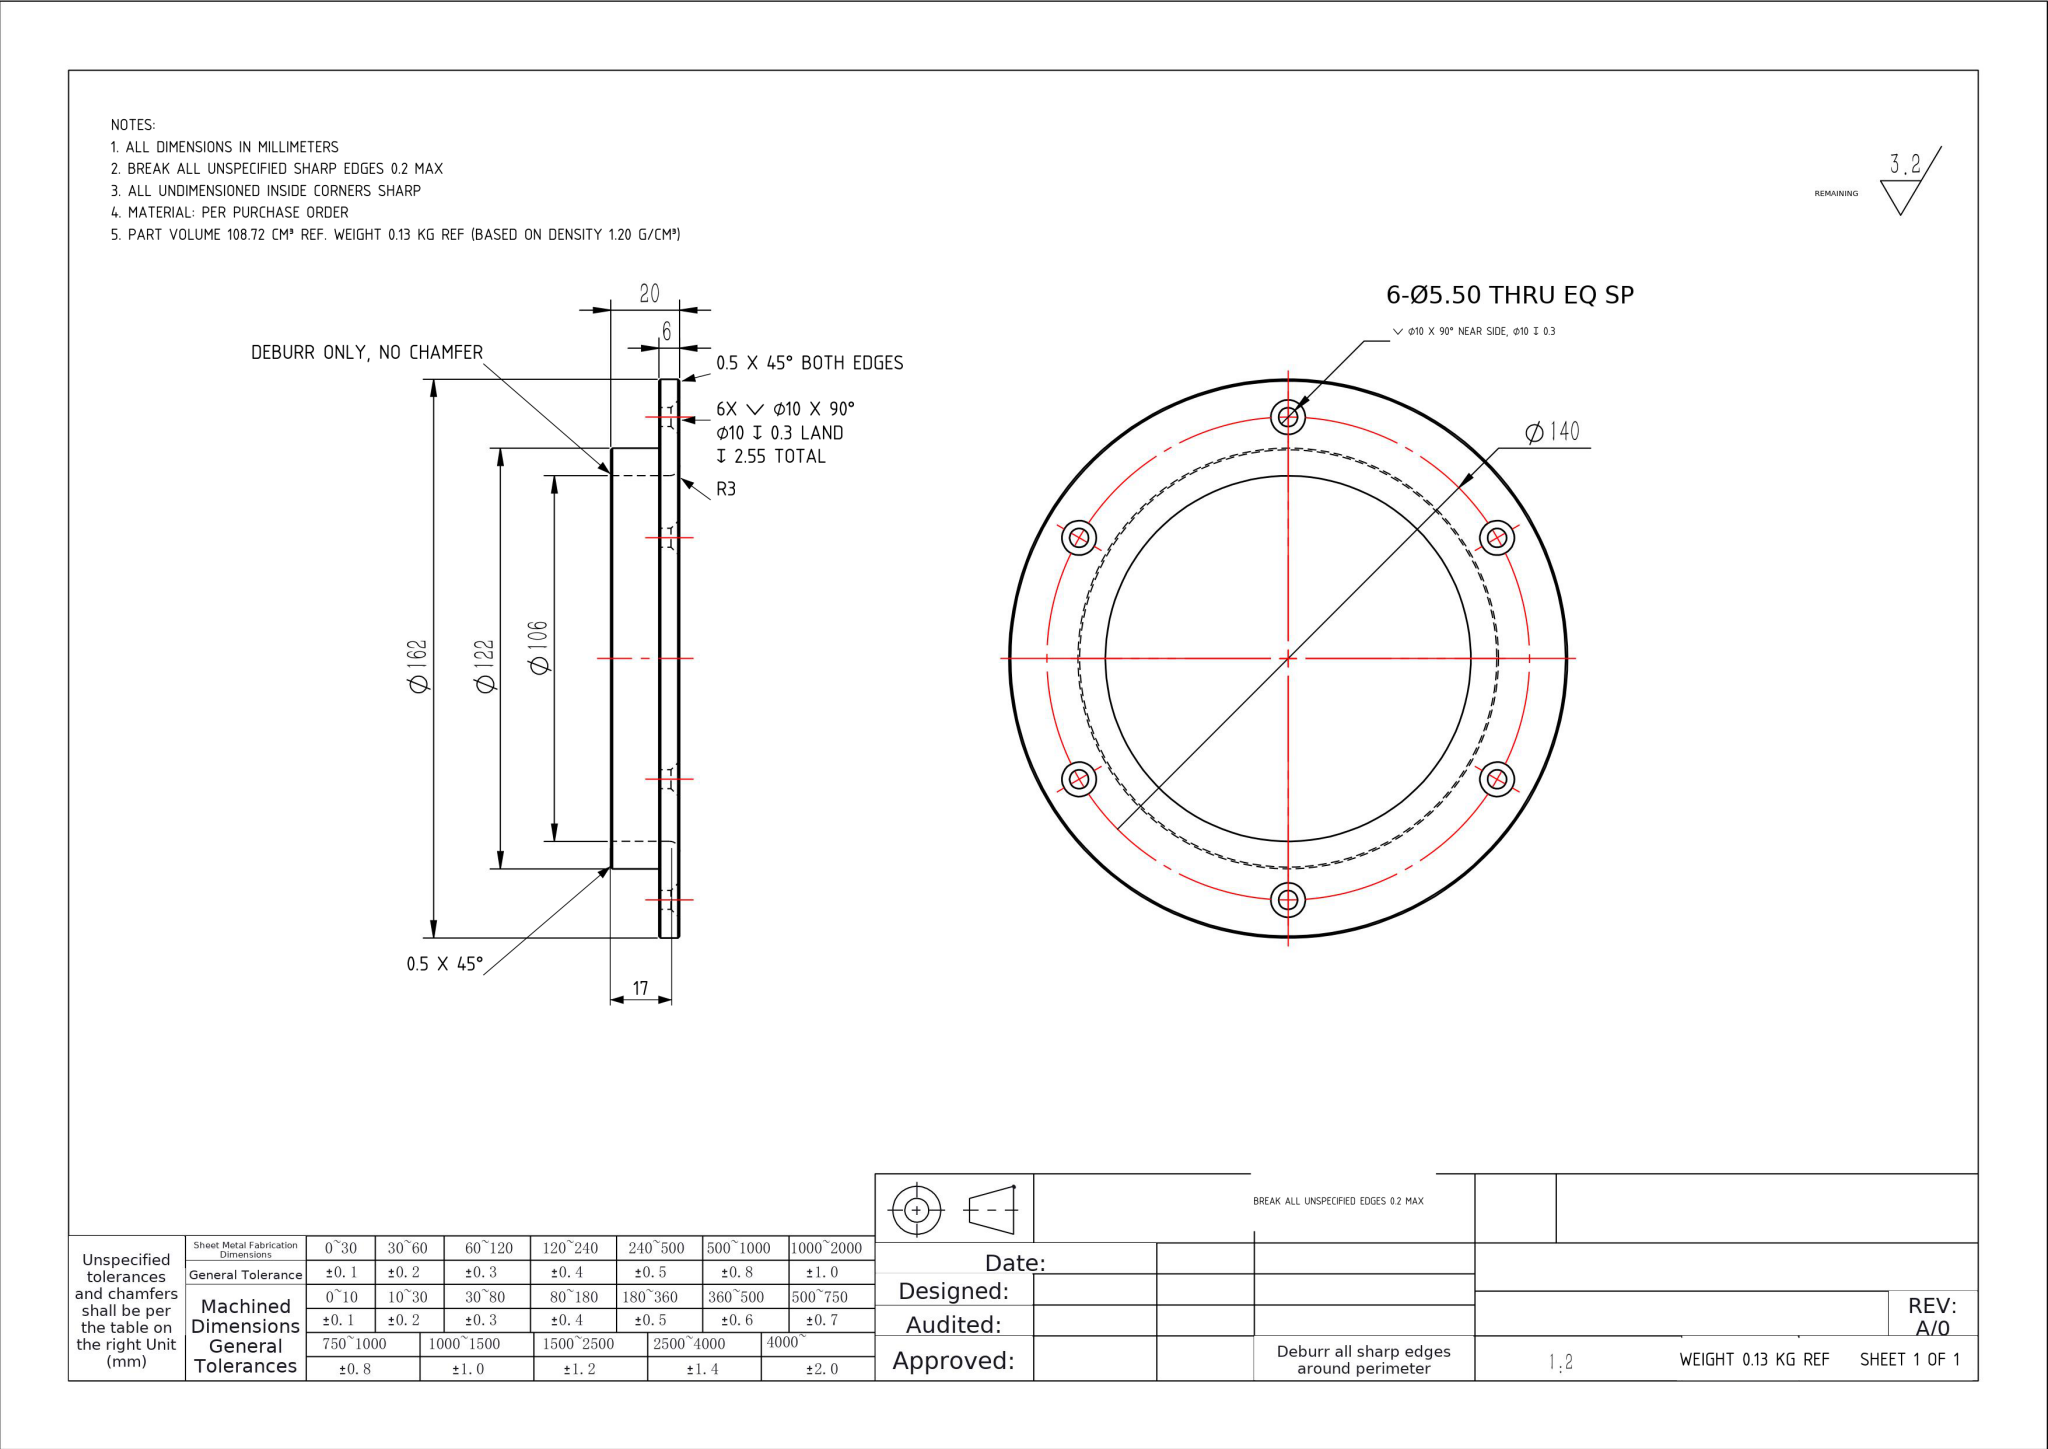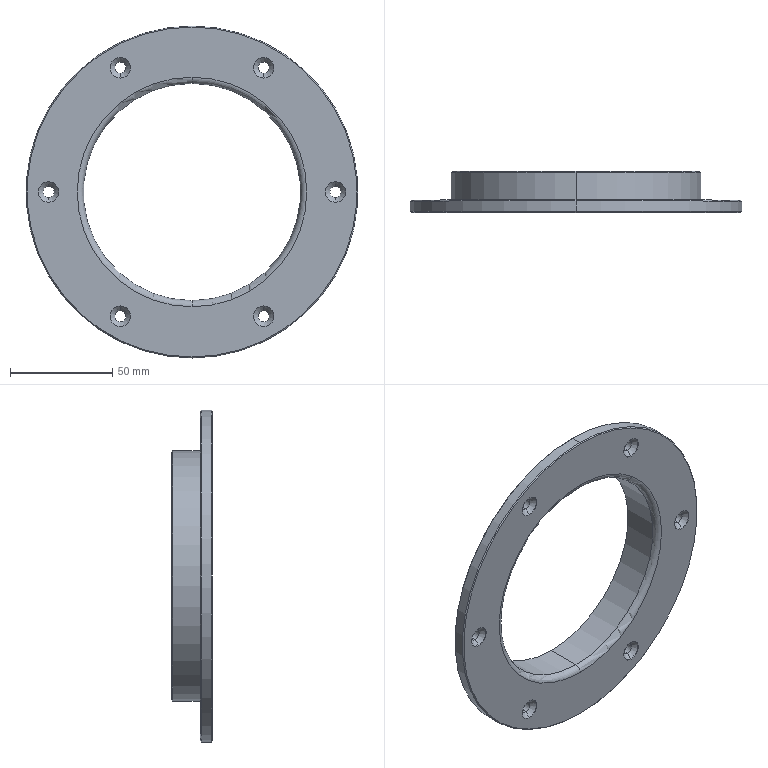Part | NX | mm | 1 solid | 53 faces | box 162 x 20 x 162 mm | volume 108721 mm3 | cylinder 30 | cone 18 | plane 3 | torus 2 | commonest cylinder face diameters 10 x12 5.5 x12 162 x2 122 x2 106 x2